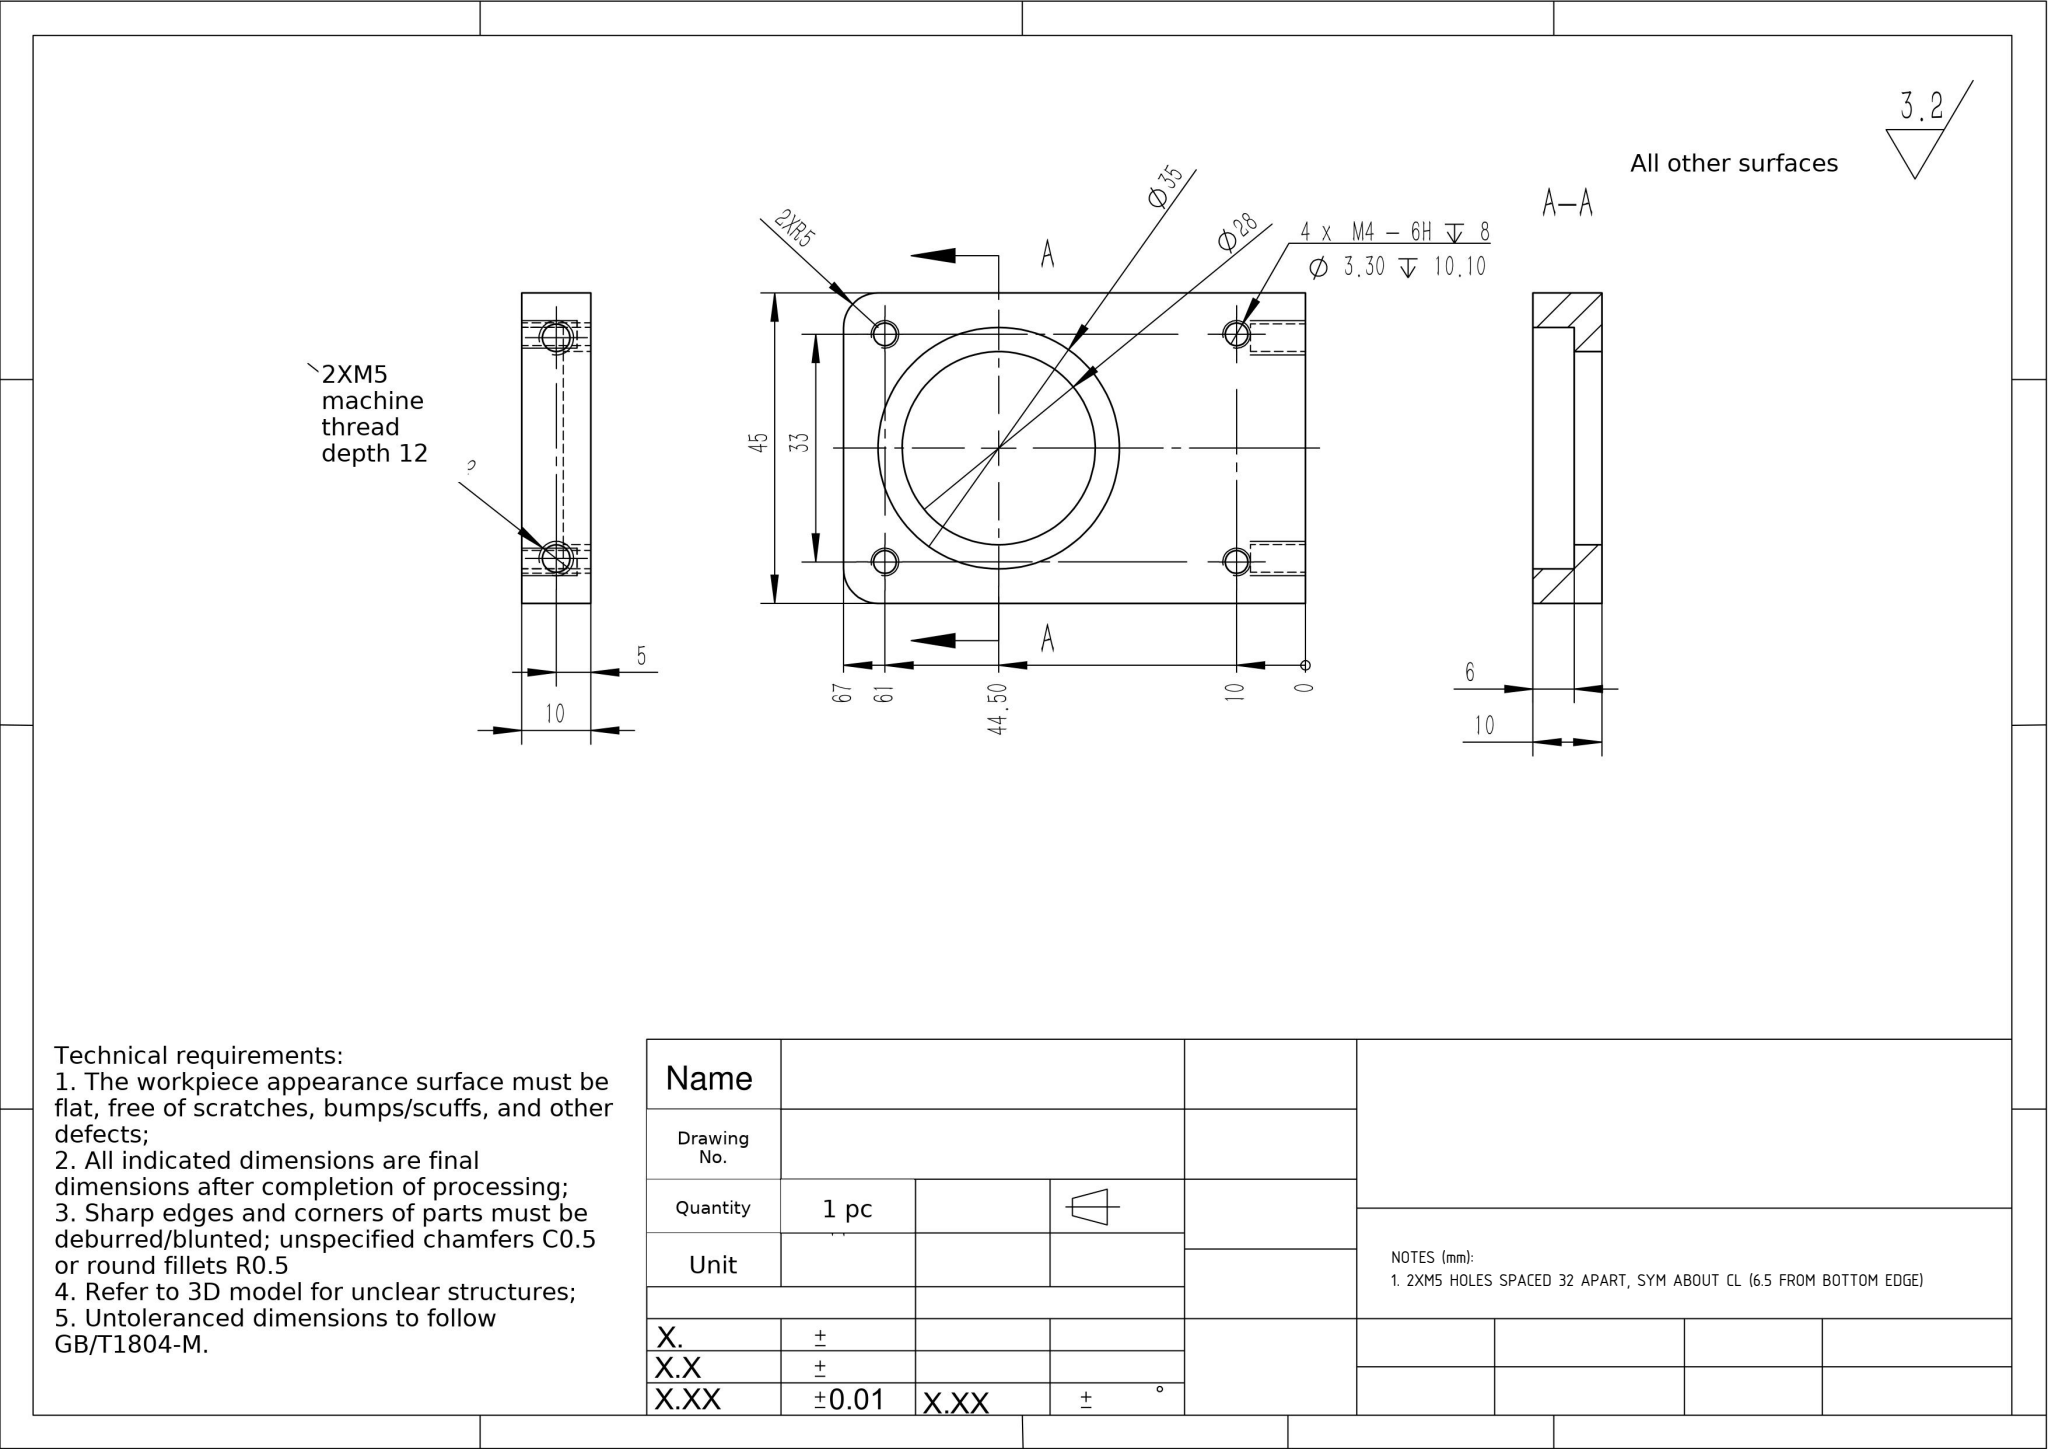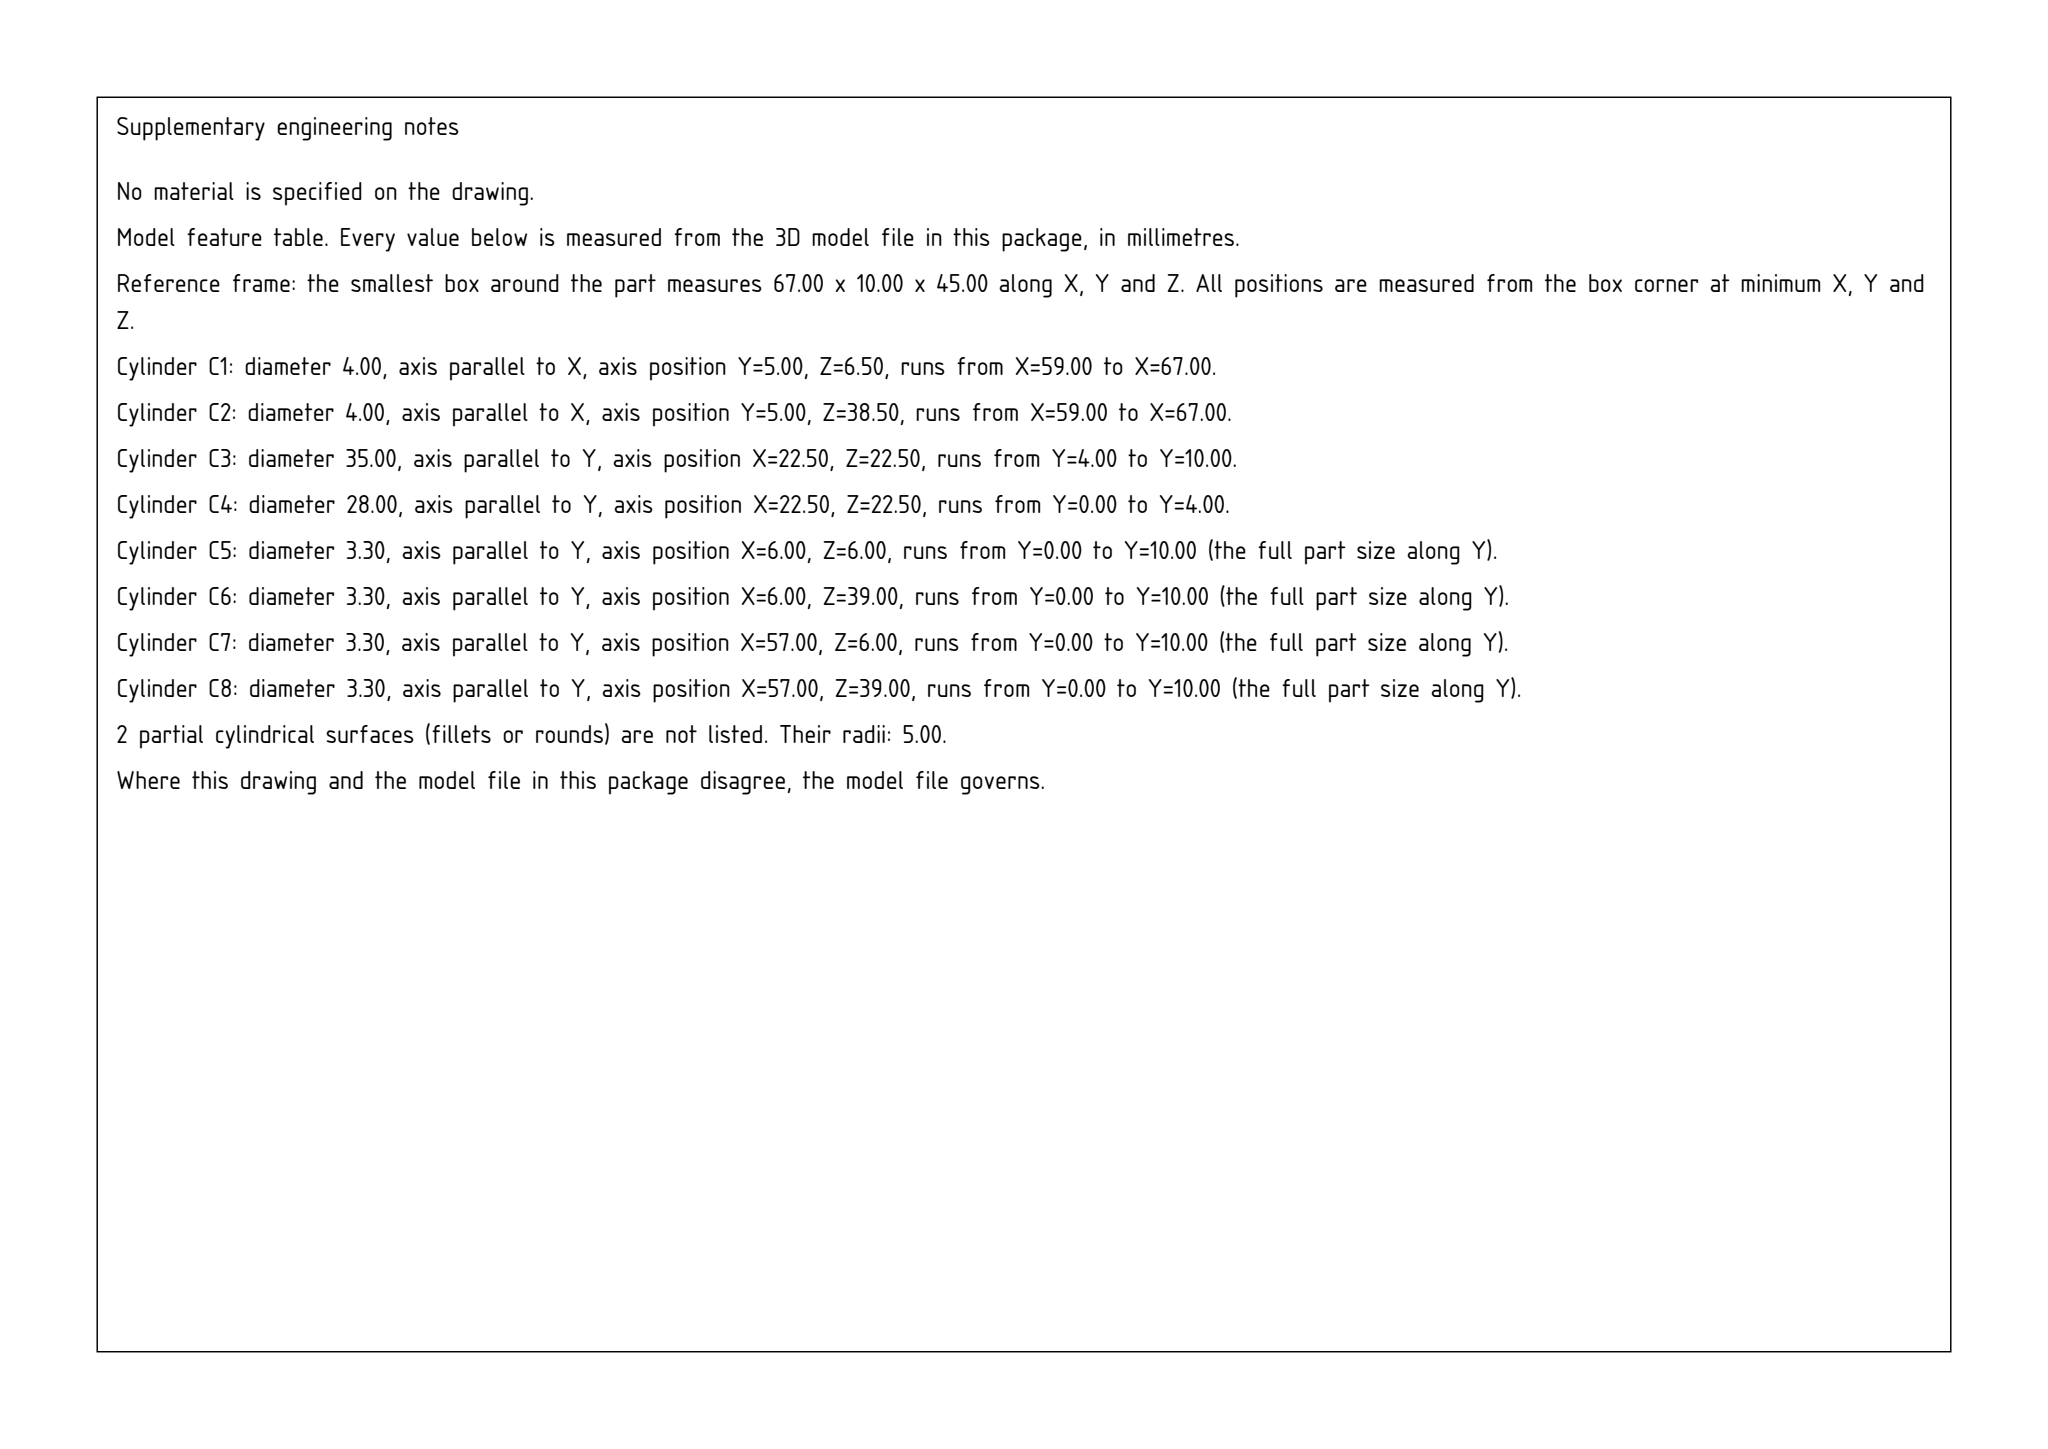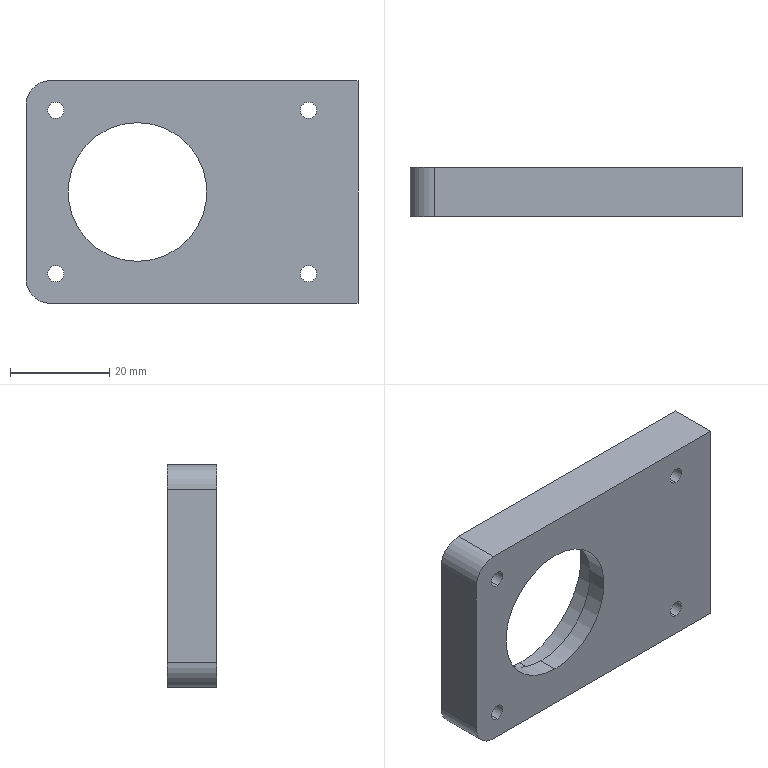Part | SolidWorks | mm | material 6061 | 1 solid | 27 faces | box 67 x 10 x 45 mm | volume 21264 mm3 | cylinder 18 | plane 9 | commonest cylinder face diameters 3.3 x8 4 x4 35 x2 28 x2 10 x2
Drawing notes:
2XM5 HOLES SPACED 32 APART, SYM ABOUT CL (6.5 FROM BOTTOM EDGE) | from the solid: Ø4 x-axis cylinders at z=6.5 and z=38.5, bbox Z=45, both at y=5.0; spacing 32, symmetric about z=22.5
build123d program:
from build123d import *

# Parameters (mm, degrees)
SKETCH1_W             = 67
SKETCH1_H             = 45
BOSS_EXTRUDE1_DEPTH   = 10
SKETCH2_R             = 14
CUT_EXTRUDE1_DEPTH    = 10
SKETCH3_R             = 17.5
CUT_EXTRUDE2_DEPTH    = 6
M4_TAPPED_HOLE1_D     = 3.3
M4_TAPPED_HOLE1_DEPTH = 10.1
M4_TAPPED_HOLE1_TIP   = 0.9914
FILLET1_R             = 5
SKETCH6_R             = 2
CUT_EXTRUDE3_DEPTH    = 8


with BuildPart() as part:
    # Sketch1 → Boss-Extrude1 (new body)
    with BuildSketch(Plane(origin=(0, 0, 0), x_dir=(1, 0, 0), z_dir=(0, 1, 0))):
        Rectangle(SKETCH1_W, SKETCH1_H)
    extrude(amount=BOSS_EXTRUDE1_DEPTH)

    # Sketch2 → Cut-Extrude1 (cut)
    with BuildSketch(Plane(origin=(0, 10, 0), x_dir=(1, 0, 0), z_dir=(0, 1, 0))):
        with Locations(Location((-11, 0, 0), (0, 0, 270))):
            Circle(SKETCH2_R)
    extrude(amount=-CUT_EXTRUDE1_DEPTH, mode=Mode.SUBTRACT)

    # Sketch3 → Cut-Extrude2 (cut)
    with BuildSketch(Plane(origin=(0, 10, 0), x_dir=(1, 0, 0), z_dir=(0, 1, 0))):
        with Locations(Location((-11, 0, 0), (0, 0, 270))):
            Circle(SKETCH3_R)
    extrude(amount=-CUT_EXTRUDE2_DEPTH, mode=Mode.SUBTRACT)

    # M4 Tapped Hole1
    with Locations(Plane(origin=(-27.5, 10, -16.5), x_dir=(0, 0, 1), z_dir=(0, 1, 0))):
        with Locations((0, 0), (33, 0), (33, 51), (0, 51)):
            Hole(M4_TAPPED_HOLE1_D / 2, depth=M4_TAPPED_HOLE1_DEPTH)
            with Locations((0, 0, -(M4_TAPPED_HOLE1_DEPTH + M4_TAPPED_HOLE1_TIP / 2))):  # 118° drill point
                Cone(0, M4_TAPPED_HOLE1_D / 2, M4_TAPPED_HOLE1_TIP, mode=Mode.SUBTRACT)

    # Fillet1
    fillet1_edges = [part.edges().sort_by_distance(p)[0] for p in [
        (-33.5, 5, 22.5),
        (-33.5, 5, -22.5),
    ]]
    fillet(fillet1_edges, radius=FILLET1_R)

    # Sketch6 → Cut-Extrude3 (cut)
    with BuildSketch(Plane(origin=(33.5, 0, 0), x_dir=(0, 0, -1), z_dir=(1, 0, 0))):
        with Locations((-16, 5)):
            Circle(SKETCH6_R)
        with Locations((16, 5)):
            Circle(SKETCH6_R)
    extrude(amount=-CUT_EXTRUDE3_DEPTH, mode=Mode.SUBTRACT)


solid = part.part
STEP:
#1=CARTESIAN_POINT('',(25.5,5.,-14.));
#2=VERTEX_POINT('',#1);
#3=CARTESIAN_POINT('',(25.5,5.,-18.));
#4=VERTEX_POINT('',#3);
#5=CARTESIAN_POINT('',(25.5,5.,-16.));
#6=DIRECTION('',(1.,0.,0.));
#7=DIRECTION('',(0.,0.,-1.));
#8=AXIS2_PLACEMENT_3D('',#5,#6,#7);
#9=CIRCLE('',#8,2.);
#10=EDGE_CURVE('',#2,#4,#9,.T.);
#11=ORIENTED_EDGE('',*,*,#10,.F.);
#12=CARTESIAN_POINT('',(33.5,5.,-14.));
#13=VERTEX_POINT('',#12);
#14=CARTESIAN_POINT('',(25.5,5.,-14.));
#15=DIRECTION('',(1.,0.,0.));
#16=VECTOR('',#15,1000.);
#17=LINE('',#14,#16);
#18=EDGE_CURVE('',#2,#13,#17,.T.);
#19=ORIENTED_EDGE('',*,*,#18,.T.);
#20=CARTESIAN_POINT('',(33.5,5.,-18.));
#21=VERTEX_POINT('',#20);
#22=CARTESIAN_POINT('',(33.5,5.,-16.));
#23=DIRECTION('',(1.,0.,0.));
#24=DIRECTION('',(0.,0.,-1.));
#25=AXIS2_PLACEMENT_3D('',#22,#23,#24);
#26=CIRCLE('',#25,2.);
#27=EDGE_CURVE('',#13,#21,#26,.T.);
#28=ORIENTED_EDGE('',*,*,#27,.T.);
#29=CARTESIAN_POINT('',(25.5,5.,-18.));
#30=DIRECTION('',(1.,0.,0.));
#31=VECTOR('',#30,1000.);
#32=LINE('',#29,#31);
#33=EDGE_CURVE('',#4,#21,#32,.T.);
#34=ORIENTED_EDGE('',*,*,#33,.F.);
#35=EDGE_LOOP('',(#11,#19,#28,#34));
#36=FACE_OUTER_BOUND('',#35,.T.);
#37=CARTESIAN_POINT('',(25.5,5.,-16.));
#38=DIRECTION('',(1.,0.,0.));
#39=DIRECTION('',(0.,0.,-1.));
#40=AXIS2_PLACEMENT_3D('',#37,#38,#39);
#41=CYLINDRICAL_SURFACE('',#40,2.);
#42=ADVANCED_FACE('',(#36),#41,.F.);
#43=CARTESIAN_POINT('',(25.5,5.,18.));
#44=VERTEX_POINT('',#43);
#45=CARTESIAN_POINT('',(25.5,5.,14.));
#46=VERTEX_POINT('',#45);
#47=CARTESIAN_POINT('',(25.5,5.,16.));
#48=DIRECTION('',(1.,0.,0.));
#49=DIRECTION('',(0.,0.,-1.));
#50=AXIS2_PLACEMENT_3D('',#47,#48,#49);
#51=CIRCLE('',#50,2.);
#52=EDGE_CURVE('',#44,#46,#51,.T.);
#53=ORIENTED_EDGE('',*,*,#52,.F.);
#54=CARTESIAN_POINT('',(33.5,5.,18.));
#55=VERTEX_POINT('',#54);
#56=CARTESIAN_POINT('',(25.5,5.,18.));
#57=DIRECTION('',(1.,0.,0.));
#58=VECTOR('',#57,1000.);
#59=LINE('',#56,#58);
#60=EDGE_CURVE('',#44,#55,#59,.T.);
#61=ORIENTED_EDGE('',*,*,#60,.T.);
#62=CARTESIAN_POINT('',(33.5,5.,14.));
#63=VERTEX_POINT('',#62);
#64=CARTESIAN_POINT('',(33.5,5.,16.));
#65=DIRECTION('',(1.,0.,0.));
#66=DIRECTION('',(0.,0.,-1.));
#67=AXIS2_PLACEMENT_3D('',#64,#65,#66);
#68=CIRCLE('',#67,2.);
#69=EDGE_CURVE('',#55,#63,#68,.T.);
#70=ORIENTED_EDGE('',*,*,#69,.T.);
#71=CARTESIAN_POINT('',(25.5,5.,14.));
#72=DIRECTION('',(1.,0.,0.));
#73=VECTOR('',#72,1000.);
#74=LINE('',#71,#73);
#75=EDGE_CURVE('',#46,#63,#74,.T.);
#76=ORIENTED_EDGE('',*,*,#75,.F.);
#77=EDGE_LOOP('',(#53,#61,#70,#76));
#78=FACE_OUTER_BOUND('',#77,.T.);
#79=CARTESIAN_POINT('',(25.5,5.,16.));
#80=DIRECTION('',(1.,0.,0.));
#81=DIRECTION('',(0.,0.,-1.));
#82=AXIS2_PLACEMENT_3D('',#79,#80,#81);
#83=CYLINDRICAL_SURFACE('',#82,2.);
#84=ADVANCED_FACE('',(#78),#83,.F.);
#85=CARTESIAN_POINT('',(-27.5,0.,-14.85));
#86=VERTEX_POINT('',#85);
#87=CARTESIAN_POINT('',(-27.5,0.,-18.15));
#88=VERTEX_POINT('',#87);
#89=CARTESIAN_POINT('',(-27.5,0.,-16.5));
#90=DIRECTION('',(0.,-1.,0.));
#91=DIRECTION('',(0.,0.,-1.));
#92=AXIS2_PLACEMENT_3D('',#89,#90,#91);
#93=CIRCLE('',#92,1.65);
#94=EDGE_CURVE('',#86,#88,#93,.T.);
#95=ORIENTED_EDGE('',*,*,#94,.T.);
#96=CARTESIAN_POINT('',(-27.5,10.,-18.15));
#97=VERTEX_POINT('',#96);
#98=CARTESIAN_POINT('',(-27.5,10.,-18.15));
#99=DIRECTION('',(0.,1.,0.));
#100=VECTOR('',#99,1000.);
#101=LINE('',#98,#100);
#102=EDGE_CURVE('',#88,#97,#101,.T.);
#103=ORIENTED_EDGE('',*,*,#102,.T.);
#104=CARTESIAN_POINT('',(-27.5,10.,-14.85));
#105=VERTEX_POINT('',#104);
#106=CARTESIAN_POINT('',(-27.5,10.,-16.5));
#107=DIRECTION('',(0.,1.,0.));
#108=DIRECTION('',(0.,0.,1.));
#109=AXIS2_PLACEMENT_3D('',#106,#107,#108);
#110=CIRCLE('',#109,1.65);
#111=EDGE_CURVE('',#97,#105,#110,.T.);
#112=ORIENTED_EDGE('',*,*,#111,.T.);
#113=CARTESIAN_POINT('',(-27.5,10.,-14.85));
#114=DIRECTION('',(0.,1.,0.));
#115=VECTOR('',#114,1000.);
#116=LINE('',#113,#115);
#117=EDGE_CURVE('',#86,#105,#116,.T.);
#118=ORIENTED_EDGE('',*,*,#117,.F.);
#119=EDGE_LOOP('',(#95,#103,#112,#118));
#120=FACE_OUTER_BOUND('',#119,.T.);
#121=CARTESIAN_POINT('',(-27.5,10.,-16.5));
#122=DIRECTION('',(0.,1.,0.));
#123=DIRECTION('',(0.,0.,1.));
#124=AXIS2_PLACEMENT_3D('',#121,#122,#123);
#125=CYLINDRICAL_SURFACE('',#124,1.65);
#126=ADVANCED_FACE('',(#120),#125,.F.);
#127=CARTESIAN_POINT('',(-27.5,0.,18.15));
#128=VERTEX_POINT('',#127);
#129=CARTESIAN_POINT('',(-27.5,0.,14.85));
#130=VERTEX_POINT('',#129);
#131=CARTESIAN_POINT('',(-27.5,0.,16.5));
#132=DIRECTION('',(0.,-1.,0.));
#133=DIRECTION('',(0.,0.,-1.));
#134=AXIS2_PLACEMENT_3D('',#131,#132,#133);
#135=CIRCLE('',#134,1.65);
#136=EDGE_CURVE('',#128,#130,#135,.T.);
#137=ORIENTED_EDGE('',*,*,#136,.T.);
#138=CARTESIAN_POINT('',(-27.5,10.,14.85));
#139=VERTEX_POINT('',#138);
#140=CARTESIAN_POINT('',(-27.5,10.,14.85));
#141=DIRECTION('',(0.,1.,0.));
#142=VECTOR('',#141,1000.);
#143=LINE('',#140,#142);
#144=EDGE_CURVE('',#130,#139,#143,.T.);
#145=ORIENTED_EDGE('',*,*,#144,.T.);
#146=CARTESIAN_POINT('',(-27.5,10.,18.15));
#147=VERTEX_POINT('',#146);
#148=CARTESIAN_POINT('',(-27.5,10.,16.5));
#149=DIRECTION('',(0.,1.,0.));
#150=DIRECTION('',(0.,0.,1.));
#151=AXIS2_PLACEMENT_3D('',#148,#149,#150);
#152=CIRCLE('',#151,1.65);
#153=EDGE_CURVE('',#139,#147,#152,.T.);
#154=ORIENTED_EDGE('',*,*,#153,.T.);
#155=CARTESIAN_POINT('',(-27.5,10.,18.15));
#156=DIRECTION('',(0.,1.,0.));
#157=VECTOR('',#156,1000.);
#158=LINE('',#155,#157);
#159=EDGE_CURVE('',#128,#147,#158,.T.);
#160=ORIENTED_EDGE('',*,*,#159,.F.);
#161=EDGE_LOOP('',(#137,#145,#154,#160));
#162=FACE_OUTER_BOUND('',#161,.T.);
#163=CARTESIAN_POINT('',(-27.5,10.,16.5));
#164=DIRECTION('',(0.,1.,0.));
#165=DIRECTION('',(0.,0.,1.));
#166=AXIS2_PLACEMENT_3D('',#163,#164,#165);
#167=CYLINDRICAL_SURFACE('',#166,1.65);
#168=ADVANCED_FACE('',(#162),#167,.F.);
#169=CARTESIAN_POINT('',(23.5,0.,18.15));
#170=VERTEX_POINT('',#169);
#171=CARTESIAN_POINT('',(23.5,0.,14.85));
#172=VERTEX_POINT('',#171);
#173=CARTESIAN_POINT('',(23.5,0.,16.5));
#174=DIRECTION('',(0.,-1.,0.));
#175=DIRECTION('',(0.,0.,-1.));
#176=AXIS2_PLACEMENT_3D('',#173,#174,#175);
#177=CIRCLE('',#176,1.65);
#178=EDGE_CURVE('',#170,#172,#177,.T.);
#179=ORIENTED_EDGE('',*,*,#178,.T.);
#180=CARTESIAN_POINT('',(23.5,10.,14.85));
#181=VERTEX_POINT('',#180);
#182=CARTESIAN_POINT('',(23.5,10.,14.85));
#183=DIRECTION('',(0.,1.,0.));
#184=VECTOR('',#183,1000.);
#185=LINE('',#182,#184);
#186=EDGE_CURVE('',#172,#181,#185,.T.);
#187=ORIENTED_EDGE('',*,*,#186,.T.);
#188=CARTESIAN_POINT('',(23.5,10.,18.15));
#189=VERTEX_POINT('',#188);
#190=CARTESIAN_POINT('',(23.5,10.,16.5));
#191=DIRECTION('',(0.,1.,0.));
#192=DIRECTION('',(0.,0.,1.));
#193=AXIS2_PLACEMENT_3D('',#190,#191,#192);
#194=CIRCLE('',#193,1.65);
#195=EDGE_CURVE('',#181,#189,#194,.T.);
#196=ORIENTED_EDGE('',*,*,#195,.T.);
#197=CARTESIAN_POINT('',(23.5,10.,18.15));
#198=DIRECTION('',(0.,1.,0.));
#199=VECTOR('',#198,1000.);
#200=LINE('',#197,#199);
#201=EDGE_CURVE('',#170,#189,#200,.T.);
#202=ORIENTED_EDGE('',*,*,#201,.F.);
#203=EDGE_LOOP('',(#179,#187,#196,#202));
#204=FACE_OUTER_BOUND('',#203,.T.);
#205=CARTESIAN_POINT('',(23.5,10.,16.5));
#206=DIRECTION('',(0.,1.,0.));
#207=DIRECTION('',(0.,0.,1.));
#208=AXIS2_PLACEMENT_3D('',#205,#206,#207);
#209=CYLINDRICAL_SURFACE('',#208,1.65);
#210=ADVANCED_FACE('',(#204),#209,.F.);
#211=CARTESIAN_POINT('',(23.5,0.,-14.85));
#212=VERTEX_POINT('',#211);
#213=CARTESIAN_POINT('',(23.5,0.,-18.15));
#214=VERTEX_POINT('',#213);
#215=CARTESIAN_POINT('',(23.5,0.,-16.5));
#216=DIRECTION('',(0.,-1.,0.));
#217=DIRECTION('',(0.,0.,-1.));
#218=AXIS2_PLACEMENT_3D('',#215,#216,#217);
#219=CIRCLE('',#218,1.65);
#220=EDGE_CURVE('',#212,#214,#219,.T.);
#221=ORIENTED_EDGE('',*,*,#220,.T.);
#222=CARTESIAN_POINT('',(23.5,10.,-18.15));
#223=VERTEX_POINT('',#222);
#224=CARTESIAN_POINT('',(23.5,10.,-18.15));
#225=DIRECTION('',(0.,1.,0.));
#226=VECTOR('',#225,1000.);
#227=LINE('',#224,#226);
#228=EDGE_CURVE('',#214,#223,#227,.T.);
#229=ORIENTED_EDGE('',*,*,#228,.T.);
#230=CARTESIAN_POINT('',(23.5,10.,-14.85));
#231=VERTEX_POINT('',#230);
#232=CARTESIAN_POINT('',(23.5,10.,-16.5));
#233=DIRECTION('',(0.,1.,0.));
#234=DIRECTION('',(0.,0.,1.));
#235=AXIS2_PLACEMENT_3D('',#232,#233,#234);
#236=CIRCLE('',#235,1.65);
#237=EDGE_CURVE('',#223,#231,#236,.T.);
#238=ORIENTED_EDGE('',*,*,#237,.T.);
#239=CARTESIAN_POINT('',(23.5,10.,-14.85));
#240=DIRECTION('',(0.,1.,0.));
#241=VECTOR('',#240,1000.);
#242=LINE('',#239,#241);
#243=EDGE_CURVE('',#212,#231,#242,.T.);
#244=ORIENTED_EDGE('',*,*,#243,.F.);
#245=EDGE_LOOP('',(#221,#229,#238,#244));
#246=FACE_OUTER_BOUND('',#245,.T.);
#247=CARTESIAN_POINT('',(23.5,10.,-16.5));
#248=DIRECTION('',(0.,1.,0.));
#249=DIRECTION('',(0.,0.,1.));
#250=AXIS2_PLACEMENT_3D('',#247,#248,#249);
#251=CYLINDRICAL_SURFACE('',#250,1.65);
#252=ADVANCED_FACE('',(#246),#251,.F.);
#253=CARTESIAN_POINT('',(-11.,4.,-17.5));
#254=VERTEX_POINT('',#253);
#255=CARTESIAN_POINT('',(-11.,4.,17.5));
#256=VERTEX_POINT('',#255);
#257=CARTESIAN_POINT('',(-11.,4.,0.));
#258=DIRECTION('',(0.,1.,0.));
#259=DIRECTION('',(0.,0.,1.));
#260=AXIS2_PLACEMENT_3D('',#257,#258,#259);
#261=CIRCLE('',#260,17.5);
#262=EDGE_CURVE('',#254,#256,#261,.T.);
#263=ORIENTED_EDGE('',*,*,#262,.F.);
#264=CARTESIAN_POINT('',(-11.,10.,-17.5));
#265=VERTEX_POINT('',#264);
#266=CARTESIAN_POINT('',(-11.,4.,-17.5));
#267=DIRECTION('',(0.,1.,0.));
#268=VECTOR('',#267,1000.);
#269=LINE('',#266,#268);
#270=EDGE_CURVE('',#254,#265,#269,.T.);
#271=ORIENTED_EDGE('',*,*,#270,.T.);
#272=CARTESIAN_POINT('',(-11.,10.,17.5));
#273=VERTEX_POINT('',#272);
#274=CARTESIAN_POINT('',(-11.,10.,0.));
#275=DIRECTION('',(0.,1.,0.));
#276=DIRECTION('',(0.,0.,1.));
#277=AXIS2_PLACEMENT_3D('',#274,#275,#276);
#278=CIRCLE('',#277,17.5);
#279=EDGE_CURVE('',#265,#273,#278,.T.);
#280=ORIENTED_EDGE('',*,*,#279,.T.);
#281=CARTESIAN_POINT('',(-11.,4.,17.5));
#282=DIRECTION('',(0.,1.,0.));
#283=VECTOR('',#282,1000.);
#284=LINE('',#281,#283);
#285=EDGE_CURVE('',#256,#273,#284,.T.);
#286=ORIENTED_EDGE('',*,*,#285,.F.);
#287=EDGE_LOOP('',(#263,#271,#280,#286));
#288=FACE_OUTER_BOUND('',#287,.T.);
#289=CARTESIAN_POINT('',(-11.,4.,0.));
#290=DIRECTION('',(0.,1.,0.));
#291=DIRECTION('',(0.,0.,1.));
#292=AXIS2_PLACEMENT_3D('',#289,#290,#291);
#293=CYLINDRICAL_SURFACE('',#292,17.5);
#294=ADVANCED_FACE('',(#288),#293,.F.);
#295=CARTESIAN_POINT('',(-11.,0.,-14.));
#296=VERTEX_POINT('',#295);
#297=CARTESIAN_POINT('',(-11.,0.,14.));
#298=VERTEX_POINT('',#297);
#299=CARTESIAN_POINT('',(-11.,0.,0.));
#300=DIRECTION('',(0.,1.,0.));
#301=DIRECTION('',(0.,0.,1.));
#302=AXIS2_PLACEMENT_3D('',#299,#300,#301);
#303=CIRCLE('',#302,14.);
#304=EDGE_CURVE('',#296,#298,#303,.T.);
#305=ORIENTED_EDGE('',*,*,#304,.F.);
#306=CARTESIAN_POINT('',(-11.,4.,-14.));
#307=VERTEX_POINT('',#306);
#308=CARTESIAN_POINT('',(-11.,0.,-14.));
#309=DIRECTION('',(0.,1.,0.));
#310=VECTOR('',#309,1000.);
#311=LINE('',#308,#310);
#312=EDGE_CURVE('',#296,#307,#311,.T.);
#313=ORIENTED_EDGE('',*,*,#312,.T.);
#314=CARTESIAN_POINT('',(-11.,4.,14.));
#315=VERTEX_POINT('',#314);
#316=CARTESIAN_POINT('',(-11.,4.,0.));
#317=DIRECTION('',(0.,-1.,0.));
#318=DIRECTION('',(0.,0.,1.));
#319=AXIS2_PLACEMENT_3D('',#316,#317,#318);
#320=CIRCLE('',#319,14.);
#321=EDGE_CURVE('',#315,#307,#320,.T.);
#322=ORIENTED_EDGE('',*,*,#321,.F.);
#323=CARTESIAN_POINT('',(-11.,0.,14.));
#324=DIRECTION('',(0.,1.,0.));
#325=VECTOR('',#324,1000.);
#326=LINE('',#323,#325);
#327=EDGE_CURVE('',#298,#315,#326,.T.);
#328=ORIENTED_EDGE('',*,*,#327,.F.);
#329=EDGE_LOOP('',(#305,#313,#322,#328));
#330=FACE_OUTER_BOUND('',#329,.T.);
#331=CARTESIAN_POINT('',(-11.,0.,0.));
#332=DIRECTION('',(0.,1.,0.));
#333=DIRECTION('',(0.,0.,1.));
#334=AXIS2_PLACEMENT_3D('',#331,#332,#333);
#335=CYLINDRICAL_SURFACE('',#334,14.);
#336=ADVANCED_FACE('',(#330),#335,.F.);
#337=ORIENTED_EDGE('',*,*,#312,.F.);
#338=CARTESIAN_POINT('',(-11.,0.,0.));
#339=DIRECTION('',(0.,1.,0.));
#340=DIRECTION('',(0.,0.,1.));
#341=AXIS2_PLACEMENT_3D('',#338,#339,#340);
#342=CIRCLE('',#341,14.);
#343=EDGE_CURVE('',#298,#296,#342,.T.);
#344=ORIENTED_EDGE('',*,*,#343,.F.);
#345=ORIENTED_EDGE('',*,*,#327,.T.);
#346=CARTESIAN_POINT('',(-11.,4.,0.));
#347=DIRECTION('',(0.,-1.,0.));
#348=DIRECTION('',(0.,0.,1.));
#349=AXIS2_PLACEMENT_3D('',#346,#347,#348);
#350=CIRCLE('',#349,14.);
#351=EDGE_CURVE('',#307,#315,#350,.T.);
#352=ORIENTED_EDGE('',*,*,#351,.F.);
#353=EDGE_LOOP('',(#337,#344,#345,#352));
#354=FACE_OUTER_BOUND('',#353,.T.);
#355=CARTESIAN_POINT('',(-11.,0.,0.));
#356=DIRECTION('',(0.,1.,0.));
#357=DIRECTION('',(0.,0.,1.));
#358=AXIS2_PLACEMENT_3D('',#355,#356,#357);
#359=CYLINDRICAL_SURFACE('',#358,14.);
#360=ADVANCED_FACE('',(#354),#359,.F.);
#361=CARTESIAN_POINT('',(33.5,5.,-16.));
#362=DIRECTION('',(1.,0.,0.));
#363=DIRECTION('',(0.,0.,-1.));
#364=AXIS2_PLACEMENT_3D('',#361,#362,#363);
#365=CIRCLE('',#364,2.);
#366=EDGE_CURVE('',#21,#13,#365,.T.);
#367=ORIENTED_EDGE('',*,*,#366,.F.);
#368=ORIENTED_EDGE('',*,*,#27,.F.);
#369=EDGE_LOOP('',(#367,#368));
#370=FACE_BOUND('',#369,.T.);
#371=CARTESIAN_POINT('',(33.5,5.,16.));
#372=DIRECTION('',(1.,0.,0.));
#373=DIRECTION('',(0.,0.,-1.));
#374=AXIS2_PLACEMENT_3D('',#371,#372,#373);
#375=CIRCLE('',#374,2.);
#376=EDGE_CURVE('',#63,#55,#375,.T.);
#377=ORIENTED_EDGE('',*,*,#376,.F.);
#378=ORIENTED_EDGE('',*,*,#69,.F.);
#379=EDGE_LOOP('',(#377,#378));
#380=FACE_BOUND('',#379,.T.);
#381=CARTESIAN_POINT('',(33.5,0.,22.5));
#382=VERTEX_POINT('',#381);
#383=CARTESIAN_POINT('',(33.5,0.,-22.5));
#384=VERTEX_POINT('',#383);
#385=CARTESIAN_POINT('',(33.5,0.,22.5));
#386=DIRECTION('',(0.,0.,-1.));
#387=VECTOR('',#386,1000.);
#388=LINE('',#385,#387);
#389=EDGE_CURVE('',#382,#384,#388,.T.);
#390=ORIENTED_EDGE('',*,*,#389,.T.);
#391=CARTESIAN_POINT('',(33.5,10.,-22.5));
#392=VERTEX_POINT('',#391);
#393=CARTESIAN_POINT('',(33.5,10.,-22.5));
#394=DIRECTION('',(0.,-1.,0.));
#395=VECTOR('',#394,1000.);
#396=LINE('',#393,#395);
#397=EDGE_CURVE('',#392,#384,#396,.T.);
#398=ORIENTED_EDGE('',*,*,#397,.F.);
#399=CARTESIAN_POINT('',(33.5,10.,22.5));
#400=VERTEX_POINT('',#399);
#401=CARTESIAN_POINT('',(33.5,10.,22.5));
#402=DIRECTION('',(0.,0.,-1.));
#403=VECTOR('',#402,1000.);
#404=LINE('',#401,#403);
#405=EDGE_CURVE('',#400,#392,#404,.T.);
#406=ORIENTED_EDGE('',*,*,#405,.F.);
#407=CARTESIAN_POINT('',(33.5,10.,22.5));
#408=DIRECTION('',(0.,-1.,0.));
#409=VECTOR('',#408,1000.);
#410=LINE('',#407,#409);
#411=EDGE_CURVE('',#400,#382,#410,.T.);
#412=ORIENTED_EDGE('',*,*,#411,.T.);
#413=EDGE_LOOP('',(#390,#398,#406,#412));
#414=FACE_OUTER_BOUND('',#413,.T.);
#415=CARTESIAN_POINT('',(33.5,10.,22.5));
#416=DIRECTION('',(-1.,0.,0.));
#417=DIRECTION('',(0.,0.,1.));
#418=AXIS2_PLACEMENT_3D('',#415,#416,#417);
#419=PLANE('',#418);
#420=ADVANCED_FACE('',(#370,#380,#414),#419,.F.);
#421=CARTESIAN_POINT('',(-28.5,0.,-22.5));
#422=VERTEX_POINT('',#421);
#423=CARTESIAN_POINT('',(-33.5,0.,-22.5));
#424=DIRECTION('',(-1.,0.,0.));
#425=VECTOR('',#424,1000.);
#426=LINE('',#423,#425);
#427=EDGE_CURVE('',#384,#422,#426,.T.);
#428=ORIENTED_EDGE('',*,*,#427,.T.);
#429=CARTESIAN_POINT('',(-28.5,10.,-22.5));
#430=VERTEX_POINT('',#429);
#431=CARTESIAN_POINT('',(-28.5,10.,-22.5));
#432=DIRECTION('',(0.,1.,0.));
#433=VECTOR('',#432,1000.);
#434=LINE('',#431,#433);
#435=EDGE_CURVE('',#422,#430,#434,.T.);
#436=ORIENTED_EDGE('',*,*,#435,.T.);
#437=CARTESIAN_POINT('',(-33.5,10.,-22.5));
#438=DIRECTION('',(-1.,0.,0.));
#439=VECTOR('',#438,1000.);
#440=LINE('',#437,#439);
#441=EDGE_CURVE('',#392,#430,#440,.T.);
#442=ORIENTED_EDGE('',*,*,#441,.F.);
#443=ORIENTED_EDGE('',*,*,#397,.T.);
#444=EDGE_LOOP('',(#428,#436,#442,#443));
#445=FACE_OUTER_BOUND('',#444,.T.);
#446=CARTESIAN_POINT('',(-33.5,10.,-22.5));
#447=DIRECTION('',(0.,0.,1.));
#448=DIRECTION('',(1.,0.,0.));
#449=AXIS2_PLACEMENT_3D('',#446,#447,#448);
#450=PLANE('',#449);
#451=ADVANCED_FACE('',(#445),#450,.F.);
#452=CARTESIAN_POINT('',(-33.5,0.,-17.5));
#453=VERTEX_POINT('',#452);
#454=CARTESIAN_POINT('',(-33.5,0.,17.5));
#455=VERTEX_POINT('',#454);
#456=CARTESIAN_POINT('',(-33.5,0.,22.5));
#457=DIRECTION('',(0.,0.,1.));
#458=VECTOR('',#457,1000.);
#459=LINE('',#456,#458);
#460=EDGE_CURVE('',#453,#455,#459,.T.);
#461=ORIENTED_EDGE('',*,*,#460,.T.);
#462=CARTESIAN_POINT('',(-33.5,10.,17.5));
#463=VERTEX_POINT('',#462);
#464=CARTESIAN_POINT('',(-33.5,10.,17.5));
#465=DIRECTION('',(0.,1.,0.));
#466=VECTOR('',#465,1000.);
#467=LINE('',#464,#466);
#468=EDGE_CURVE('',#455,#463,#467,.T.);
#469=ORIENTED_EDGE('',*,*,#468,.T.);
#470=CARTESIAN_POINT('',(-33.5,10.,-17.5));
#471=VERTEX_POINT('',#470);
#472=CARTESIAN_POINT('',(-33.5,10.,22.5));
#473=DIRECTION('',(0.,0.,1.));
#474=VECTOR('',#473,1000.);
#475=LINE('',#472,#474);
#476=EDGE_CURVE('',#471,#463,#475,.T.);
#477=ORIENTED_EDGE('',*,*,#476,.F.);
#478=CARTESIAN_POINT('',(-33.5,10.,-17.5));
#479=DIRECTION('',(0.,-1.,0.));
#480=VECTOR('',#479,1000.);
#481=LINE('',#478,#480);
#482=EDGE_CURVE('',#471,#453,#481,.T.);
#483=ORIENTED_EDGE('',*,*,#482,.T.);
#484=EDGE_LOOP('',(#461,#469,#477,#483));
#485=FACE_OUTER_BOUND('',#484,.T.);
#486=CARTESIAN_POINT('',(-33.5,10.,22.5));
#487=DIRECTION('',(1.,0.,0.));
#488=DIRECTION('',(0.,0.,-1.));
#489=AXIS2_PLACEMENT_3D('',#486,#487,#488);
#490=PLANE('',#489);
#491=ADVANCED_FACE('',(#485),#490,.F.);
#492=CARTESIAN_POINT('',(-28.5,10.,22.5));
#493=VERTEX_POINT('',#492);
#494=CARTESIAN_POINT('',(-33.5,10.,22.5));
#495=DIRECTION('',(1.,0.,0.));
#496=VECTOR('',#495,1000.);
#497=LINE('',#494,#496);
#498=EDGE_CURVE('',#493,#400,#497,.T.);
#499=ORIENTED_EDGE('',*,*,#498,.F.);
#500=CARTESIAN_POINT('',(-28.5,0.,22.5));
#501=VERTEX_POINT('',#500);
#502=CARTESIAN_POINT('',(-28.5,10.,22.5));
#503=DIRECTION('',(0.,-1.,0.));
#504=VECTOR('',#503,1000.);
#505=LINE('',#502,#504);
#506=EDGE_CURVE('',#493,#501,#505,.T.);
#507=ORIENTED_EDGE('',*,*,#506,.T.);
#508=CARTESIAN_POINT('',(-33.5,0.,22.5));
#509=DIRECTION('',(1.,0.,0.));
#510=VECTOR('',#509,1000.);
#511=LINE('',#508,#510);
#512=EDGE_CURVE('',#501,#382,#511,.T.);
#513=ORIENTED_EDGE('',*,*,#512,.T.);
#514=ORIENTED_EDGE('',*,*,#411,.F.);
#515=EDGE_LOOP('',(#499,#507,#513,#514));
#516=FACE_OUTER_BOUND('',#515,.T.);
#517=CARTESIAN_POINT('',(-33.5,10.,22.5));
#518=DIRECTION('',(0.,0.,-1.));
#519=DIRECTION('',(-1.,0.,0.));
#520=AXIS2_PLACEMENT_3D('',#517,#518,#519);
#521=PLANE('',#520);
#522=ADVANCED_FACE('',(#516),#521,.F.);
#523=CARTESIAN_POINT('',(-27.5,10.,-16.5));
#524=DIRECTION('',(0.,1.,0.));
#525=DIRECTION('',(0.,0.,1.));
#526=AXIS2_PLACEMENT_3D('',#523,#524,#525);
#527=CIRCLE('',#526,1.65);
#528=EDGE_CURVE('',#105,#97,#527,.T.);
#529=ORIENTED_EDGE('',*,*,#528,.F.);
#530=ORIENTED_EDGE('',*,*,#111,.F.);
#531=EDGE_LOOP('',(#529,#530));
#532=FACE_BOUND('',#531,.T.);
#533=CARTESIAN_POINT('',(-27.5,10.,16.5));
#534=DIRECTION('',(0.,1.,0.));
#535=DIRECTION('',(0.,0.,1.));
#536=AXIS2_PLACEMENT_3D('',#533,#534,#535);
#537=CIRCLE('',#536,1.65);
#538=EDGE_CURVE('',#147,#139,#537,.T.);
#539=ORIENTED_EDGE('',*,*,#538,.F.);
#540=ORIENTED_EDGE('',*,*,#153,.F.);
#541=EDGE_LOOP('',(#539,#540));
#542=FACE_BOUND('',#541,.T.);
#543=CARTESIAN_POINT('',(23.5,10.,16.5));
#544=DIRECTION('',(0.,1.,0.));
#545=DIRECTION('',(0.,0.,1.));
#546=AXIS2_PLACEMENT_3D('',#543,#544,#545);
#547=CIRCLE('',#546,1.65);
#548=EDGE_CURVE('',#189,#181,#547,.T.);
#549=ORIENTED_EDGE('',*,*,#548,.F.);
#550=ORIENTED_EDGE('',*,*,#195,.F.);
#551=EDGE_LOOP('',(#549,#550));
#552=FACE_BOUND('',#551,.T.);
#553=CARTESIAN_POINT('',(23.5,10.,-16.5));
#554=DIRECTION('',(0.,1.,0.));
#555=DIRECTION('',(0.,0.,1.));
#556=AXIS2_PLACEMENT_3D('',#553,#554,#555);
#557=CIRCLE('',#556,1.65);
#558=EDGE_CURVE('',#231,#223,#557,.T.);
#559=ORIENTED_EDGE('',*,*,#558,.F.);
#560=ORIENTED_EDGE('',*,*,#237,.F.);
#561=EDGE_LOOP('',(#559,#560));
#562=FACE_BOUND('',#561,.T.);
#563=CARTESIAN_POINT('',(-11.,10.,0.));
#564=DIRECTION('',(0.,1.,0.));
#565=DIRECTION('',(0.,0.,1.));
#566=AXIS2_PLACEMENT_3D('',#563,#564,#565);
#567=CIRCLE('',#566,17.5);
#568=EDGE_CURVE('',#273,#265,#567,.T.);
#569=ORIENTED_EDGE('',*,*,#568,.F.);
#570=ORIENTED_EDGE('',*,*,#279,.F.);
#571=EDGE_LOOP('',(#569,#570));
#572=FACE_BOUND('',#571,.T.);
#573=ORIENTED_EDGE('',*,*,#476,.T.);
#574=CARTESIAN_POINT('',(-28.5,10.,17.5));
#575=DIRECTION('',(0.,1.,0.));
#576=DIRECTION('',(0.,0.,-1.));
#577=AXIS2_PLACEMENT_3D('',#574,#575,#576);
#578=CIRCLE('',#577,5.);
#579=EDGE_CURVE('',#463,#493,#578,.T.);
#580=ORIENTED_EDGE('',*,*,#579,.T.);
#581=ORIENTED_EDGE('',*,*,#498,.T.);
#582=ORIENTED_EDGE('',*,*,#405,.T.);
#583=ORIENTED_EDGE('',*,*,#441,.T.);
#584=CARTESIAN_POINT('',(-28.5,10.,-17.5));
#585=DIRECTION('',(0.,1.,0.));
#586=DIRECTION('',(0.,0.,-1.));
#587=AXIS2_PLACEMENT_3D('',#584,#585,#586);
#588=CIRCLE('',#587,5.);
#589=EDGE_CURVE('',#430,#471,#588,.T.);
#590=ORIENTED_EDGE('',*,*,#589,.T.);
#591=EDGE_LOOP('',(#573,#580,#581,#582,#583,#590));
#592=FACE_OUTER_BOUND('',#591,.T.);
#593=CARTESIAN_POINT('',(0.,10.,0.));
#594=DIRECTION('',(0.,-1.,0.));
#595=DIRECTION('',(0.,0.,-1.));
#596=AXIS2_PLACEMENT_3D('',#593,#594,#595);
#597=PLANE('',#596);
#598=ADVANCED_FACE('',(#532,#542,#552,#562,#572,#592),#597,.F.);
#599=ORIENTED_EDGE('',*,*,#94,.F.);
#600=CARTESIAN_POINT('',(-27.5,0.,-16.5));
#601=DIRECTION('',(0.,-1.,0.));
#602=DIRECTION('',(0.,0.,-1.));
#603=AXIS2_PLACEMENT_3D('',#600,#601,#602);
#604=CIRCLE('',#603,1.65);
#605=EDGE_CURVE('',#88,#86,#604,.T.);
#606=ORIENTED_EDGE('',*,*,#605,.F.);
#607=EDGE_LOOP('',(#599,#606));
#608=FACE_BOUND('',#607,.T.);
#609=ORIENTED_EDGE('',*,*,#136,.F.);
#610=CARTESIAN_POINT('',(-27.5,0.,16.5));
#611=DIRECTION('',(0.,-1.,0.));
#612=DIRECTION('',(0.,0.,-1.));
#613=AXIS2_PLACEMENT_3D('',#610,#611,#612);
#614=CIRCLE('',#613,1.65);
#615=EDGE_CURVE('',#130,#128,#614,.T.);
#616=ORIENTED_EDGE('',*,*,#615,.F.);
#617=EDGE_LOOP('',(#609,#616));
#618=FACE_BOUND('',#617,.T.);
#619=ORIENTED_EDGE('',*,*,#178,.F.);
#620=CARTESIAN_POINT('',(23.5,0.,16.5));
#621=DIRECTION('',(0.,-1.,0.));
#622=DIRECTION('',(0.,0.,-1.));
#623=AXIS2_PLACEMENT_3D('',#620,#621,#622);
#624=CIRCLE('',#623,1.65);
#625=EDGE_CURVE('',#172,#170,#624,.T.);
#626=ORIENTED_EDGE('',*,*,#625,.F.);
#627=EDGE_LOOP('',(#619,#626));
#628=FACE_BOUND('',#627,.T.);
#629=ORIENTED_EDGE('',*,*,#220,.F.);
#630=CARTESIAN_POINT('',(23.5,0.,-16.5));
#631=DIRECTION('',(0.,-1.,0.));
#632=DIRECTION('',(0.,0.,-1.));
#633=AXIS2_PLACEMENT_3D('',#630,#631,#632);
#634=CIRCLE('',#633,1.65);
#635=EDGE_CURVE('',#214,#212,#634,.T.);
#636=ORIENTED_EDGE('',*,*,#635,.F.);
#637=EDGE_LOOP('',(#629,#636));
#638=FACE_BOUND('',#637,.T.);
#639=ORIENTED_EDGE('',*,*,#343,.T.);
#640=ORIENTED_EDGE('',*,*,#304,.T.);
#641=EDGE_LOOP('',(#639,#640));
#642=FACE_BOUND('',#641,.T.);
#643=ORIENTED_EDGE('',*,*,#512,.F.);
#644=CARTESIAN_POINT('',(-28.5,0.,17.5));
#645=DIRECTION('',(0.,-1.,0.));
#646=DIRECTION('',(0.,0.,-1.));
#647=AXIS2_PLACEMENT_3D('',#644,#645,#646);
#648=CIRCLE('',#647,5.);
#649=EDGE_CURVE('',#501,#455,#648,.T.);
#650=ORIENTED_EDGE('',*,*,#649,.T.);
#651=ORIENTED_EDGE('',*,*,#460,.F.);
#652=CARTESIAN_POINT('',(-28.5,0.,-17.5));
#653=DIRECTION('',(0.,-1.,0.));
#654=DIRECTION('',(0.,0.,-1.));
#655=AXIS2_PLACEMENT_3D('',#652,#653,#654);
#656=CIRCLE('',#655,5.);
#657=EDGE_CURVE('',#453,#422,#656,.T.);
#658=ORIENTED_EDGE('',*,*,#657,.T.);
#659=ORIENTED_EDGE('',*,*,#427,.F.);
#660=ORIENTED_EDGE('',*,*,#389,.F.);
#661=EDGE_LOOP('',(#643,#650,#651,#658,#659,#660));
#662=FACE_OUTER_BOUND('',#661,.T.);
#663=CARTESIAN_POINT('',(0.,0.,0.));
#664=DIRECTION('',(0.,-1.,0.));
#665=DIRECTION('',(0.,0.,-1.));
#666=AXIS2_PLACEMENT_3D('',#663,#664,#665);
#667=PLANE('',#666);
#668=ADVANCED_FACE('',(#608,#618,#628,#638,#642,#662),#667,.T.);
#669=CARTESIAN_POINT('',(-11.,4.,0.));
#670=DIRECTION('',(0.,1.,0.));
#671=DIRECTION('',(0.,0.,1.));
#672=AXIS2_PLACEMENT_3D('',#669,#670,#671);
#673=CIRCLE('',#672,17.5);
#674=EDGE_CURVE('',#256,#254,#673,.T.);
#675=ORIENTED_EDGE('',*,*,#674,.T.);
#676=ORIENTED_EDGE('',*,*,#262,.T.);
#677=EDGE_LOOP('',(#675,#676));
#678=FACE_OUTER_BOUND('',#677,.T.);
#679=ORIENTED_EDGE('',*,*,#321,.T.);
#680=ORIENTED_EDGE('',*,*,#351,.T.);
#681=EDGE_LOOP('',(#679,#680));
#682=FACE_BOUND('',#681,.T.);
#683=CARTESIAN_POINT('',(-11.,4.,0.));
#684=DIRECTION('',(0.,1.,0.));
#685=DIRECTION('',(0.,0.,1.));
#686=AXIS2_PLACEMENT_3D('',#683,#684,#685);
#687=PLANE('',#686);
#688=ADVANCED_FACE('',(#678,#682),#687,.T.);
#689=ORIENTED_EDGE('',*,*,#270,.F.);
#690=ORIENTED_EDGE('',*,*,#674,.F.);
#691=ORIENTED_EDGE('',*,*,#285,.T.);
#692=ORIENTED_EDGE('',*,*,#568,.T.);
#693=EDGE_LOOP('',(#689,#690,#691,#692));
#694=FACE_OUTER_BOUND('',#693,.T.);
#695=CARTESIAN_POINT('',(-11.,4.,0.));
#696=DIRECTION('',(0.,1.,0.));
#697=DIRECTION('',(0.,0.,1.));
#698=AXIS2_PLACEMENT_3D('',#695,#696,#697);
#699=CYLINDRICAL_SURFACE('',#698,17.5);
#700=ADVANCED_FACE('',(#694),#699,.F.);
#701=ORIENTED_EDGE('',*,*,#228,.F.);
#702=ORIENTED_EDGE('',*,*,#635,.T.);
#703=ORIENTED_EDGE('',*,*,#243,.T.);
#704=ORIENTED_EDGE('',*,*,#558,.T.);
#705=EDGE_LOOP('',(#701,#702,#703,#704));
#706=FACE_OUTER_BOUND('',#705,.T.);
#707=CARTESIAN_POINT('',(23.5,10.,-16.5));
#708=DIRECTION('',(0.,1.,0.));
#709=DIRECTION('',(0.,0.,1.));
#710=AXIS2_PLACEMENT_3D('',#707,#708,#709);
#711=CYLINDRICAL_SURFACE('',#710,1.65);
#712=ADVANCED_FACE('',(#706),#711,.F.);
#713=ORIENTED_EDGE('',*,*,#186,.F.);
#714=ORIENTED_EDGE('',*,*,#625,.T.);
#715=ORIENTED_EDGE('',*,*,#201,.T.);
#716=ORIENTED_EDGE('',*,*,#548,.T.);
#717=EDGE_LOOP('',(#713,#714,#715,#716));
#718=FACE_OUTER_BOUND('',#717,.T.);
#719=CARTESIAN_POINT('',(23.5,10.,16.5));
#720=DIRECTION('',(0.,1.,0.));
#721=DIRECTION('',(0.,0.,1.));
#722=AXIS2_PLACEMENT_3D('',#719,#720,#721);
#723=CYLINDRICAL_SURFACE('',#722,1.65);
#724=ADVANCED_FACE('',(#718),#723,.F.);
#725=ORIENTED_EDGE('',*,*,#144,.F.);
#726=ORIENTED_EDGE('',*,*,#615,.T.);
#727=ORIENTED_EDGE('',*,*,#159,.T.);
#728=ORIENTED_EDGE('',*,*,#538,.T.);
#729=EDGE_LOOP('',(#725,#726,#727,#728));
#730=FACE_OUTER_BOUND('',#729,.T.);
#731=CARTESIAN_POINT('',(-27.5,10.,16.5));
#732=DIRECTION('',(0.,1.,0.));
#733=DIRECTION('',(0.,0.,1.));
#734=AXIS2_PLACEMENT_3D('',#731,#732,#733);
#735=CYLINDRICAL_SURFACE('',#734,1.65);
#736=ADVANCED_FACE('',(#730),#735,.F.);
#737=ORIENTED_EDGE('',*,*,#102,.F.);
#738=ORIENTED_EDGE('',*,*,#605,.T.);
#739=ORIENTED_EDGE('',*,*,#117,.T.);
#740=ORIENTED_EDGE('',*,*,#528,.T.);
#741=EDGE_LOOP('',(#737,#738,#739,#740));
#742=FACE_OUTER_BOUND('',#741,.T.);
#743=CARTESIAN_POINT('',(-27.5,10.,-16.5));
#744=DIRECTION('',(0.,1.,0.));
#745=DIRECTION('',(0.,0.,1.));
#746=AXIS2_PLACEMENT_3D('',#743,#744,#745);
#747=CYLINDRICAL_SURFACE('',#746,1.65);
#748=ADVANCED_FACE('',(#742),#747,.F.);
#749=ORIENTED_EDGE('',*,*,#579,.F.);
#750=ORIENTED_EDGE('',*,*,#468,.F.);
#751=ORIENTED_EDGE('',*,*,#649,.F.);
#752=ORIENTED_EDGE('',*,*,#506,.F.);
#753=EDGE_LOOP('',(#749,#750,#751,#752));
#754=FACE_OUTER_BOUND('',#753,.T.);
#755=CARTESIAN_POINT('',(-28.5,10.,17.5));
#756=DIRECTION('',(0.,-1.,0.));
#757=DIRECTION('',(0.,0.,-1.));
#758=AXIS2_PLACEMENT_3D('',#755,#756,#757);
#759=CYLINDRICAL_SURFACE('',#758,5.);
#760=ADVANCED_FACE('',(#754),#759,.T.);
#761=ORIENTED_EDGE('',*,*,#589,.F.);
#762=ORIENTED_EDGE('',*,*,#435,.F.);
#763=ORIENTED_EDGE('',*,*,#657,.F.);
#764=ORIENTED_EDGE('',*,*,#482,.F.);
#765=EDGE_LOOP('',(#761,#762,#763,#764));
#766=FACE_OUTER_BOUND('',#765,.T.);
#767=CARTESIAN_POINT('',(-28.5,10.,-17.5));
#768=DIRECTION('',(0.,-1.,0.));
#769=DIRECTION('',(0.,0.,-1.));
#770=AXIS2_PLACEMENT_3D('',#767,#768,#769);
#771=CYLINDRICAL_SURFACE('',#770,5.);
#772=ADVANCED_FACE('',(#766),#771,.T.);
#773=ORIENTED_EDGE('',*,*,#60,.F.);
#774=CARTESIAN_POINT('',(25.5,5.,16.));
#775=DIRECTION('',(1.,0.,0.));
#776=DIRECTION('',(0.,0.,-1.));
#777=AXIS2_PLACEMENT_3D('',#774,#775,#776);
#778=CIRCLE('',#777,2.);
#779=EDGE_CURVE('',#46,#44,#778,.T.);
#780=ORIENTED_EDGE('',*,*,#779,.F.);
#781=ORIENTED_EDGE('',*,*,#75,.T.);
#782=ORIENTED_EDGE('',*,*,#376,.T.);
#783=EDGE_LOOP('',(#773,#780,#781,#782));
#784=FACE_OUTER_BOUND('',#783,.T.);
#785=CARTESIAN_POINT('',(25.5,5.,16.));
#786=DIRECTION('',(1.,0.,0.));
#787=DIRECTION('',(0.,0.,-1.));
#788=AXIS2_PLACEMENT_3D('',#785,#786,#787);
#789=CYLINDRICAL_SURFACE('',#788,2.);
#790=ADVANCED_FACE('',(#784),#789,.F.);
#791=ORIENTED_EDGE('',*,*,#779,.T.);
#792=ORIENTED_EDGE('',*,*,#52,.T.);
#793=EDGE_LOOP('',(#791,#792));
#794=FACE_OUTER_BOUND('',#793,.T.);
#795=CARTESIAN_POINT('',(25.5,5.,16.));
#796=DIRECTION('',(1.,0.,0.));
#797=DIRECTION('',(0.,0.,-1.));
#798=AXIS2_PLACEMENT_3D('',#795,#796,#797);
#799=PLANE('',#798);
#800=ADVANCED_FACE('',(#794),#799,.T.);
#801=ORIENTED_EDGE('',*,*,#18,.F.);
#802=CARTESIAN_POINT('',(25.5,5.,-16.));
#803=DIRECTION('',(1.,0.,0.));
#804=DIRECTION('',(0.,0.,-1.));
#805=AXIS2_PLACEMENT_3D('',#802,#803,#804);
#806=CIRCLE('',#805,2.);
#807=EDGE_CURVE('',#4,#2,#806,.T.);
#808=ORIENTED_EDGE('',*,*,#807,.F.);
#809=ORIENTED_EDGE('',*,*,#33,.T.);
#810=ORIENTED_EDGE('',*,*,#366,.T.);
#811=EDGE_LOOP('',(#801,#808,#809,#810));
#812=FACE_OUTER_BOUND('',#811,.T.);
#813=CARTESIAN_POINT('',(25.5,5.,-16.));
#814=DIRECTION('',(1.,0.,0.));
#815=DIRECTION('',(0.,0.,-1.));
#816=AXIS2_PLACEMENT_3D('',#813,#814,#815);
#817=CYLINDRICAL_SURFACE('',#816,2.);
#818=ADVANCED_FACE('',(#812),#817,.F.);
#819=ORIENTED_EDGE('',*,*,#807,.T.);
#820=ORIENTED_EDGE('',*,*,#10,.T.);
#821=EDGE_LOOP('',(#819,#820));
#822=FACE_OUTER_BOUND('',#821,.T.);
#823=CARTESIAN_POINT('',(25.5,5.,-16.));
#824=DIRECTION('',(1.,0.,0.));
#825=DIRECTION('',(0.,0.,-1.));
#826=AXIS2_PLACEMENT_3D('',#823,#824,#825);
#827=PLANE('',#826);
#828=ADVANCED_FACE('',(#822),#827,.T.);
#829=CLOSED_SHELL('',(#42,#84,#126,#168,#210,#252,#294,#336,#360,#420,#451,#491,#522,#598,#668,#688,#700,#712,#724,#736,#748,#760,#772,#790,#800,#818,#828));
#830=MANIFOLD_SOLID_BREP('',#829);
#831=CARTESIAN_POINT('',(0.,0.,0.));
#832=DIRECTION('',(0.,0.,1.));
#833=DIRECTION('',(1.,0.,0.));
#834=AXIS2_PLACEMENT_3D('',#831,#832,#833);
#835=(LENGTH_UNIT()NAMED_UNIT(*)SI_UNIT(.MILLI.,.METRE.));
#836=UNCERTAINTY_MEASURE_WITH_UNIT(LENGTH_MEASURE(0.00001),#835,'','');
#837=(NAMED_UNIT(*)PLANE_ANGLE_UNIT()SI_UNIT($,.RADIAN.));
#838=(NAMED_UNIT(*)SI_UNIT($,.STERADIAN.)SOLID_ANGLE_UNIT());
#839=(GEOMETRIC_REPRESENTATION_CONTEXT(3)GLOBAL_UNCERTAINTY_ASSIGNED_CONTEXT((#836))GLOBAL_UNIT_ASSIGNED_CONTEXT((#835,#837,#838))REPRESENTATION_CONTEXT('',''));
#840=ADVANCED_BREP_SHAPE_REPRESENTATION('',(#830,#834),#839);